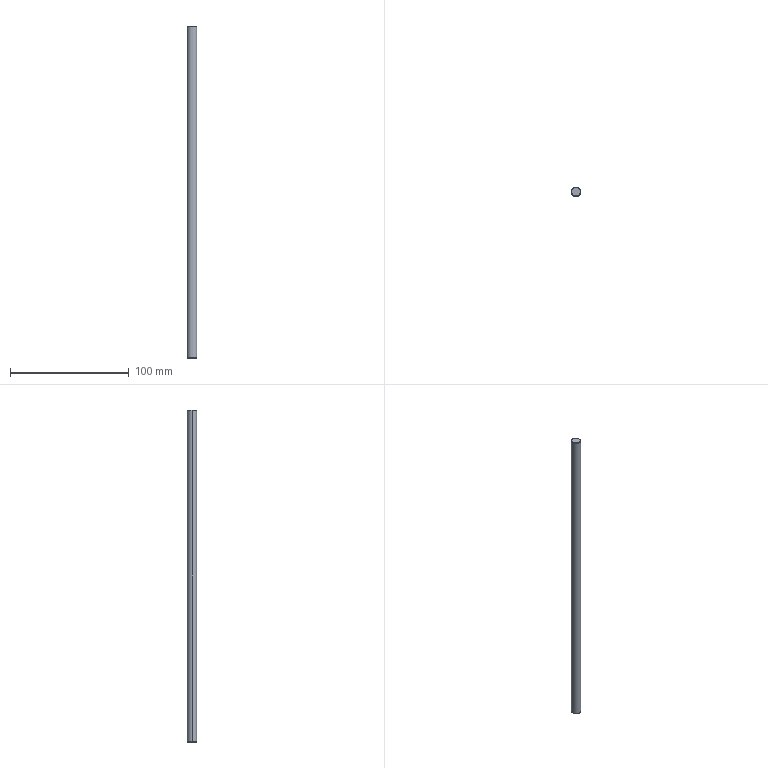Component | SolidWorks | LD101-02--Q1020-Q1-2-1 | 1 solid | 12 faces | box 8 x 8 x 280 mm | volume 13863 mm3 | cone 6 | cylinder 4 | plane 2 | commonest cylinder face diameters 4.2 x2 8 x2 | material 45
build123d program:
from build123d import *

# Parameters (mm, degrees)
SKETCH1_R             = 4
BOSS_EXTRUDE1_DEPTH   = 140
CHAMFER1_SIZE         = 0.5
M5_TAPPED_HOLE1_D     = 4.2
M5_TAPPED_HOLE1_DEPTH = 14.4
M5_TAPPED_HOLE1_TIP   = 1.262


with BuildPart() as part:
    # Sketch1 → Boss-Extrude1 (new, symmetric)
    with BuildSketch(Plane.XY):
        Circle(SKETCH1_R)
    extrude(amount=BOSS_EXTRUDE1_DEPTH, both=True)

    # Chamfer1
    chamfer1_edges = [part.edges().sort_by_distance(p)[0] for p in [
        (-4, 0, -140),
        (-4, 0, 140),
    ]]
    chamfer(chamfer1_edges, length=CHAMFER1_SIZE)

    # M5 Tapped Hole1
    with Locations(Plane(origin=(0, 0, -140), x_dir=(1, 0, 0), z_dir=(0, 0, -1))):
        with Locations((0, 0)):
            Hole(M5_TAPPED_HOLE1_D / 2, depth=M5_TAPPED_HOLE1_DEPTH)
            with Locations((0, 0, -(M5_TAPPED_HOLE1_DEPTH + M5_TAPPED_HOLE1_TIP / 2))):  # 118° drill point
                Cone(0, M5_TAPPED_HOLE1_D / 2, M5_TAPPED_HOLE1_TIP, mode=Mode.SUBTRACT)


solid = part.part

# Placed as in the assembly
solid = solid.moved(Location((-440.29, -154.897, 139.257), (0, 0, 0)))
STEP:
#1=COLOUR_RGB('',0.7922,0.8196,0.9333);
#2=FILL_AREA_STYLE_COLOUR('',#1);
#3=FILL_AREA_STYLE('',(#2));
#4=SURFACE_STYLE_FILL_AREA(#3);
#5=SURFACE_SIDE_STYLE('',(#4));
#6=SURFACE_STYLE_USAGE(.BOTH.,#5);
#7=PRESENTATION_STYLE_ASSIGNMENT((#6));
#8=CARTESIAN_POINT('',(-17.252,-6.098,0.5377));
#9=VERTEX_POINT('',#8);
#10=CARTESIAN_POINT('',(-17.417,-6.098,0.5377));
#11=VERTEX_POINT('',#10);
#12=CARTESIAN_POINT('',(-17.334,-6.098,0.5377));
#13=DIRECTION('',(0.,0.,-1.));
#14=DIRECTION('',(-1.,0.,0.));
#15=AXIS2_PLACEMENT_3D('',#12,#13,#14);
#16=CIRCLE('',#15,0.08268);
#17=EDGE_CURVE('',#9,#11,#16,.T.);
#18=ORIENTED_EDGE('',*,*,#17,.F.);
#19=CARTESIAN_POINT('',(-17.252,-6.098,-0.02927));
#20=VERTEX_POINT('',#19);
#21=CARTESIAN_POINT('',(-17.252,-6.098,-0.02927));
#22=DIRECTION('',(0.,0.,-1.));
#23=VECTOR('',#22,39.37);
#24=LINE('',#21,#23);
#25=EDGE_CURVE('',#9,#20,#24,.T.);
#26=ORIENTED_EDGE('',*,*,#25,.T.);
#27=CARTESIAN_POINT('',(-17.417,-6.098,-0.02927));
#28=VERTEX_POINT('',#27);
#29=CARTESIAN_POINT('',(-17.334,-6.098,-0.02927));
#30=DIRECTION('',(0.,0.,-1.));
#31=DIRECTION('',(-1.,0.,0.));
#32=AXIS2_PLACEMENT_3D('',#29,#30,#31);
#33=CIRCLE('',#32,0.08268);
#34=EDGE_CURVE('',#20,#28,#33,.T.);
#35=ORIENTED_EDGE('',*,*,#34,.T.);
#36=CARTESIAN_POINT('',(-17.417,-6.098,-0.02927));
#37=DIRECTION('',(0.,0.,-1.));
#38=VECTOR('',#37,39.37);
#39=LINE('',#36,#38);
#40=EDGE_CURVE('',#11,#28,#39,.T.);
#41=ORIENTED_EDGE('',*,*,#40,.F.);
#42=EDGE_LOOP('',(#18,#26,#35,#41));
#43=FACE_OUTER_BOUND('',#42,.T.);
#44=CARTESIAN_POINT('',(-17.334,-6.098,-0.02927));
#45=DIRECTION('',(0.,0.,-1.));
#46=DIRECTION('',(-1.,0.,0.));
#47=AXIS2_PLACEMENT_3D('',#44,#45,#46);
#48=CYLINDRICAL_SURFACE('',#47,0.08268);
#49=ADVANCED_FACE('',(#43),#48,.F.);
#50=CARTESIAN_POINT('',(-17.334,-6.098,0.5873));
#51=VERTEX_POINT('',#50);
#52=CARTESIAN_POINT('',(-17.417,-6.098,0.5377));
#53=DIRECTION('',(-0.8572,0.,-0.515));
#54=VECTOR('',#53,39.37);
#55=LINE('',#52,#54);
#56=EDGE_CURVE('',#51,#11,#55,.T.);
#57=ORIENTED_EDGE('',*,*,#56,.F.);
#58=CARTESIAN_POINT('',(-17.252,-6.098,0.5377));
#59=DIRECTION('',(0.8572,0.,-0.515));
#60=VECTOR('',#59,39.37);
#61=LINE('',#58,#60);
#62=EDGE_CURVE('',#51,#9,#61,.T.);
#63=ORIENTED_EDGE('',*,*,#62,.T.);
#64=ORIENTED_EDGE('',*,*,#17,.T.);
#65=EDGE_LOOP('',(#57,#63,#64));
#66=FACE_OUTER_BOUND('',#65,.T.);
#67=CARTESIAN_POINT('',(-17.334,-6.098,0.5377));
#68=DIRECTION('',(0.,0.,-1.));
#69=DIRECTION('',(-1.,0.,0.));
#70=AXIS2_PLACEMENT_3D('',#67,#68,#69);
#71=CONICAL_SURFACE('',#70,0.08268,1.03);
#72=ADVANCED_FACE('',(#66),#71,.F.);
#73=CARTESIAN_POINT('',(-17.196,-6.098,10.994));
#74=VERTEX_POINT('',#73);
#75=CARTESIAN_POINT('',(-17.472,-6.098,10.994));
#76=VERTEX_POINT('',#75);
#77=CARTESIAN_POINT('',(-17.334,-6.098,10.994));
#78=DIRECTION('',(0.,0.,1.));
#79=DIRECTION('',(1.,0.,0.));
#80=AXIS2_PLACEMENT_3D('',#77,#78,#79);
#81=CIRCLE('',#80,0.1378);
#82=EDGE_CURVE('',#74,#76,#81,.T.);
#83=ORIENTED_EDGE('',*,*,#82,.F.);
#84=CARTESIAN_POINT('',(-17.177,-6.098,10.975));
#85=VERTEX_POINT('',#84);
#86=CARTESIAN_POINT('',(-17.196,-6.098,10.994));
#87=DIRECTION('',(0.7071,0.,-0.7071));
#88=VECTOR('',#87,39.37);
#89=LINE('',#86,#88);
#90=EDGE_CURVE('',#74,#85,#89,.T.);
#91=ORIENTED_EDGE('',*,*,#90,.T.);
#92=CARTESIAN_POINT('',(-17.492,-6.098,10.975));
#93=VERTEX_POINT('',#92);
#94=CARTESIAN_POINT('',(-17.334,-6.098,10.975));
#95=DIRECTION('',(0.,0.,-1.));
#96=DIRECTION('',(1.,0.,0.));
#97=AXIS2_PLACEMENT_3D('',#94,#95,#96);
#98=CIRCLE('',#97,0.1575);
#99=EDGE_CURVE('',#93,#85,#98,.T.);
#100=ORIENTED_EDGE('',*,*,#99,.F.);
#101=CARTESIAN_POINT('',(-17.472,-6.098,10.994));
#102=DIRECTION('',(-0.7071,0.,-0.7071));
#103=VECTOR('',#102,39.37);
#104=LINE('',#101,#103);
#105=EDGE_CURVE('',#76,#93,#104,.T.);
#106=ORIENTED_EDGE('',*,*,#105,.F.);
#107=EDGE_LOOP('',(#83,#91,#100,#106));
#108=FACE_OUTER_BOUND('',#107,.T.);
#109=CARTESIAN_POINT('',(-17.334,-6.098,10.994));
#110=DIRECTION('',(0.,0.,-1.));
#111=DIRECTION('',(-1.,0.,0.));
#112=AXIS2_PLACEMENT_3D('',#109,#110,#111);
#113=CONICAL_SURFACE('',#112,0.1378,0.7854);
#114=ADVANCED_FACE('',(#108),#113,.T.);
#115=CARTESIAN_POINT('',(-17.472,-6.098,-0.02927));
#116=VERTEX_POINT('',#115);
#117=CARTESIAN_POINT('',(-17.196,-6.098,-0.02927));
#118=VERTEX_POINT('',#117);
#119=CARTESIAN_POINT('',(-17.334,-6.098,-0.02927));
#120=DIRECTION('',(0.,0.,-1.));
#121=DIRECTION('',(1.,0.,0.));
#122=AXIS2_PLACEMENT_3D('',#119,#120,#121);
#123=CIRCLE('',#122,0.1378);
#124=EDGE_CURVE('',#116,#118,#123,.T.);
#125=ORIENTED_EDGE('',*,*,#124,.F.);
#126=CARTESIAN_POINT('',(-17.492,-6.098,-0.009581));
#127=VERTEX_POINT('',#126);
#128=CARTESIAN_POINT('',(-17.492,-6.098,-0.009581));
#129=DIRECTION('',(-0.7071,0.,0.7071));
#130=VECTOR('',#129,39.37);
#131=LINE('',#128,#130);
#132=EDGE_CURVE('',#116,#127,#131,.T.);
#133=ORIENTED_EDGE('',*,*,#132,.T.);
#134=CARTESIAN_POINT('',(-17.177,-6.098,-0.009581));
#135=VERTEX_POINT('',#134);
#136=CARTESIAN_POINT('',(-17.334,-6.098,-0.009581));
#137=DIRECTION('',(0.,0.,1.));
#138=DIRECTION('',(1.,0.,0.));
#139=AXIS2_PLACEMENT_3D('',#136,#137,#138);
#140=CIRCLE('',#139,0.1575);
#141=EDGE_CURVE('',#135,#127,#140,.T.);
#142=ORIENTED_EDGE('',*,*,#141,.F.);
#143=CARTESIAN_POINT('',(-17.177,-6.098,-0.009581));
#144=DIRECTION('',(0.7071,0.,0.7071));
#145=VECTOR('',#144,39.37);
#146=LINE('',#143,#145);
#147=EDGE_CURVE('',#118,#135,#146,.T.);
#148=ORIENTED_EDGE('',*,*,#147,.F.);
#149=EDGE_LOOP('',(#125,#133,#142,#148));
#150=FACE_OUTER_BOUND('',#149,.T.);
#151=CARTESIAN_POINT('',(-17.334,-6.098,-0.009581));
#152=DIRECTION('',(0.,0.,1.));
#153=DIRECTION('',(1.,0.,0.));
#154=AXIS2_PLACEMENT_3D('',#151,#152,#153);
#155=CONICAL_SURFACE('',#154,0.1575,0.7854);
#156=ADVANCED_FACE('',(#150),#155,.T.);
#157=ORIENTED_EDGE('',*,*,#99,.T.);
#158=CARTESIAN_POINT('',(-17.177,-6.098,10.994));
#159=DIRECTION('',(0.,0.,-1.));
#160=VECTOR('',#159,39.37);
#161=LINE('',#158,#160);
#162=EDGE_CURVE('',#85,#135,#161,.T.);
#163=ORIENTED_EDGE('',*,*,#162,.T.);
#164=ORIENTED_EDGE('',*,*,#141,.T.);
#165=CARTESIAN_POINT('',(-17.492,-6.098,10.994));
#166=DIRECTION('',(0.,0.,-1.));
#167=VECTOR('',#166,39.37);
#168=LINE('',#165,#167);
#169=EDGE_CURVE('',#93,#127,#168,.T.);
#170=ORIENTED_EDGE('',*,*,#169,.F.);
#171=EDGE_LOOP('',(#157,#163,#164,#170));
#172=FACE_OUTER_BOUND('',#171,.T.);
#173=CARTESIAN_POINT('',(-17.334,-6.098,10.994));
#174=DIRECTION('',(0.,0.,-1.));
#175=DIRECTION('',(-1.,0.,0.));
#176=AXIS2_PLACEMENT_3D('',#173,#174,#175);
#177=CYLINDRICAL_SURFACE('',#176,0.1575);
#178=ADVANCED_FACE('',(#172),#177,.T.);
#179=ORIENTED_EDGE('',*,*,#162,.F.);
#180=CARTESIAN_POINT('',(-17.334,-6.098,10.975));
#181=DIRECTION('',(0.,0.,-1.));
#182=DIRECTION('',(1.,0.,0.));
#183=AXIS2_PLACEMENT_3D('',#180,#181,#182);
#184=CIRCLE('',#183,0.1575);
#185=EDGE_CURVE('',#85,#93,#184,.T.);
#186=ORIENTED_EDGE('',*,*,#185,.T.);
#187=ORIENTED_EDGE('',*,*,#169,.T.);
#188=CARTESIAN_POINT('',(-17.334,-6.098,-0.009581));
#189=DIRECTION('',(0.,0.,1.));
#190=DIRECTION('',(1.,0.,0.));
#191=AXIS2_PLACEMENT_3D('',#188,#189,#190);
#192=CIRCLE('',#191,0.1575);
#193=EDGE_CURVE('',#127,#135,#192,.T.);
#194=ORIENTED_EDGE('',*,*,#193,.T.);
#195=EDGE_LOOP('',(#179,#186,#187,#194));
#196=FACE_OUTER_BOUND('',#195,.T.);
#197=CARTESIAN_POINT('',(-17.334,-6.098,10.994));
#198=DIRECTION('',(0.,0.,-1.));
#199=DIRECTION('',(-1.,0.,0.));
#200=AXIS2_PLACEMENT_3D('',#197,#198,#199);
#201=CYLINDRICAL_SURFACE('',#200,0.1575);
#202=ADVANCED_FACE('',(#196),#201,.T.);
#203=CARTESIAN_POINT('',(-17.334,-6.098,10.994));
#204=DIRECTION('',(0.,0.,1.));
#205=DIRECTION('',(1.,0.,0.));
#206=AXIS2_PLACEMENT_3D('',#203,#204,#205);
#207=CIRCLE('',#206,0.1378);
#208=EDGE_CURVE('',#76,#74,#207,.T.);
#209=ORIENTED_EDGE('',*,*,#208,.T.);
#210=ORIENTED_EDGE('',*,*,#82,.T.);
#211=EDGE_LOOP('',(#209,#210));
#212=FACE_OUTER_BOUND('',#211,.T.);
#213=CARTESIAN_POINT('',(-17.334,-6.098,10.994));
#214=DIRECTION('',(0.,0.,1.));
#215=DIRECTION('',(1.,0.,0.));
#216=AXIS2_PLACEMENT_3D('',#213,#214,#215);
#217=PLANE('',#216);
#218=ADVANCED_FACE('',(#212),#217,.T.);
#219=CARTESIAN_POINT('',(-17.334,-6.098,-0.02927));
#220=DIRECTION('',(0.,0.,-1.));
#221=DIRECTION('',(-1.,0.,0.));
#222=AXIS2_PLACEMENT_3D('',#219,#220,#221);
#223=CIRCLE('',#222,0.08268);
#224=EDGE_CURVE('',#28,#20,#223,.T.);
#225=ORIENTED_EDGE('',*,*,#224,.F.);
#226=ORIENTED_EDGE('',*,*,#34,.F.);
#227=EDGE_LOOP('',(#225,#226));
#228=FACE_BOUND('',#227,.T.);
#229=CARTESIAN_POINT('',(-17.334,-6.098,-0.02927));
#230=DIRECTION('',(0.,0.,-1.));
#231=DIRECTION('',(1.,0.,0.));
#232=AXIS2_PLACEMENT_3D('',#229,#230,#231);
#233=CIRCLE('',#232,0.1378);
#234=EDGE_CURVE('',#118,#116,#233,.T.);
#235=ORIENTED_EDGE('',*,*,#234,.T.);
#236=ORIENTED_EDGE('',*,*,#124,.T.);
#237=EDGE_LOOP('',(#235,#236));
#238=FACE_OUTER_BOUND('',#237,.T.);
#239=CARTESIAN_POINT('',(-17.334,-6.098,-0.02927));
#240=DIRECTION('',(0.,0.,1.));
#241=DIRECTION('',(1.,0.,0.));
#242=AXIS2_PLACEMENT_3D('',#239,#240,#241);
#243=PLANE('',#242);
#244=ADVANCED_FACE('',(#228,#238),#243,.F.);
#245=ORIENTED_EDGE('',*,*,#132,.F.);
#246=ORIENTED_EDGE('',*,*,#234,.F.);
#247=ORIENTED_EDGE('',*,*,#147,.T.);
#248=ORIENTED_EDGE('',*,*,#193,.F.);
#249=EDGE_LOOP('',(#245,#246,#247,#248));
#250=FACE_OUTER_BOUND('',#249,.T.);
#251=CARTESIAN_POINT('',(-17.334,-6.098,-0.009581));
#252=DIRECTION('',(0.,0.,1.));
#253=DIRECTION('',(1.,0.,0.));
#254=AXIS2_PLACEMENT_3D('',#251,#252,#253);
#255=CONICAL_SURFACE('',#254,0.1575,0.7854);
#256=ADVANCED_FACE('',(#250),#255,.T.);
#257=ORIENTED_EDGE('',*,*,#90,.F.);
#258=ORIENTED_EDGE('',*,*,#208,.F.);
#259=ORIENTED_EDGE('',*,*,#105,.T.);
#260=ORIENTED_EDGE('',*,*,#185,.F.);
#261=EDGE_LOOP('',(#257,#258,#259,#260));
#262=FACE_OUTER_BOUND('',#261,.T.);
#263=CARTESIAN_POINT('',(-17.334,-6.098,10.994));
#264=DIRECTION('',(0.,0.,-1.));
#265=DIRECTION('',(-1.,0.,0.));
#266=AXIS2_PLACEMENT_3D('',#263,#264,#265);
#267=CONICAL_SURFACE('',#266,0.1378,0.7854);
#268=ADVANCED_FACE('',(#262),#267,.T.);
#269=ORIENTED_EDGE('',*,*,#62,.F.);
#270=ORIENTED_EDGE('',*,*,#56,.T.);
#271=CARTESIAN_POINT('',(-17.334,-6.098,0.5377));
#272=DIRECTION('',(0.,0.,-1.));
#273=DIRECTION('',(-1.,0.,0.));
#274=AXIS2_PLACEMENT_3D('',#271,#272,#273);
#275=CIRCLE('',#274,0.08268);
#276=EDGE_CURVE('',#11,#9,#275,.T.);
#277=ORIENTED_EDGE('',*,*,#276,.T.);
#278=EDGE_LOOP('',(#269,#270,#277));
#279=FACE_OUTER_BOUND('',#278,.T.);
#280=CARTESIAN_POINT('',(-17.334,-6.098,0.5377));
#281=DIRECTION('',(0.,0.,-1.));
#282=DIRECTION('',(-1.,0.,0.));
#283=AXIS2_PLACEMENT_3D('',#280,#281,#282);
#284=CONICAL_SURFACE('',#283,0.08268,1.03);
#285=ADVANCED_FACE('',(#279),#284,.F.);
#286=ORIENTED_EDGE('',*,*,#25,.F.);
#287=ORIENTED_EDGE('',*,*,#276,.F.);
#288=ORIENTED_EDGE('',*,*,#40,.T.);
#289=ORIENTED_EDGE('',*,*,#224,.T.);
#290=EDGE_LOOP('',(#286,#287,#288,#289));
#291=FACE_OUTER_BOUND('',#290,.T.);
#292=CARTESIAN_POINT('',(-17.334,-6.098,-0.02927));
#293=DIRECTION('',(0.,0.,-1.));
#294=DIRECTION('',(-1.,0.,0.));
#295=AXIS2_PLACEMENT_3D('',#292,#293,#294);
#296=CYLINDRICAL_SURFACE('',#295,0.08268);
#297=ADVANCED_FACE('',(#291),#296,.F.);
#298=CLOSED_SHELL('',(#49,#72,#114,#156,#178,#202,#218,#244,#256,#268,#285,#297));
#299=MANIFOLD_SOLID_BREP('',#298);
#300=STYLED_ITEM('',(#7),#299);
#301=PRESENTATION_LAYER_ASSIGNMENT('','',(#300));
#302=(LENGTH_UNIT()NAMED_UNIT(*)SI_UNIT($,.METRE.));
#303=LENGTH_MEASURE_WITH_UNIT(LENGTH_MEASURE(0.0254),#302);
#304=DIMENSIONAL_EXPONENTS(1.,0.,0.,0.,0.,0.,0.);
#305=(CONVERSION_BASED_UNIT('',#303)LENGTH_UNIT()NAMED_UNIT(#304));
#306=UNCERTAINTY_MEASURE_WITH_UNIT(LENGTH_MEASURE(0.00001),#305,'','');
#307=(NAMED_UNIT(*)PLANE_ANGLE_UNIT()SI_UNIT($,.RADIAN.));
#308=(NAMED_UNIT(*)SI_UNIT($,.STERADIAN.)SOLID_ANGLE_UNIT());
#309=(GEOMETRIC_REPRESENTATION_CONTEXT(3)GLOBAL_UNCERTAINTY_ASSIGNED_CONTEXT((#306))GLOBAL_UNIT_ASSIGNED_CONTEXT((#305,#307,#308))REPRESENTATION_CONTEXT('',''));
#310=MECHANICAL_DESIGN_GEOMETRIC_PRESENTATION_REPRESENTATION('',(#300),#309);
#311=CARTESIAN_POINT('',(0.,0.,0.));
#312=DIRECTION('',(0.,0.,1.));
#313=DIRECTION('',(1.,0.,0.));
#314=AXIS2_PLACEMENT_3D('',#311,#312,#313);
#315=(LENGTH_UNIT()NAMED_UNIT(*)SI_UNIT($,.METRE.));
#316=LENGTH_MEASURE_WITH_UNIT(LENGTH_MEASURE(0.0254),#315);
#317=DIMENSIONAL_EXPONENTS(1.,0.,0.,0.,0.,0.,0.);
#318=(CONVERSION_BASED_UNIT('',#316)LENGTH_UNIT()NAMED_UNIT(#317));
#319=UNCERTAINTY_MEASURE_WITH_UNIT(LENGTH_MEASURE(0.00001),#318,'','');
#320=(NAMED_UNIT(*)PLANE_ANGLE_UNIT()SI_UNIT($,.RADIAN.));
#321=(NAMED_UNIT(*)SI_UNIT($,.STERADIAN.)SOLID_ANGLE_UNIT());
#322=(GEOMETRIC_REPRESENTATION_CONTEXT(3)GLOBAL_UNCERTAINTY_ASSIGNED_CONTEXT((#319))GLOBAL_UNIT_ASSIGNED_CONTEXT((#318,#320,#321))REPRESENTATION_CONTEXT('',''));
#323=ADVANCED_BREP_SHAPE_REPRESENTATION('',(#299,#314),#322);